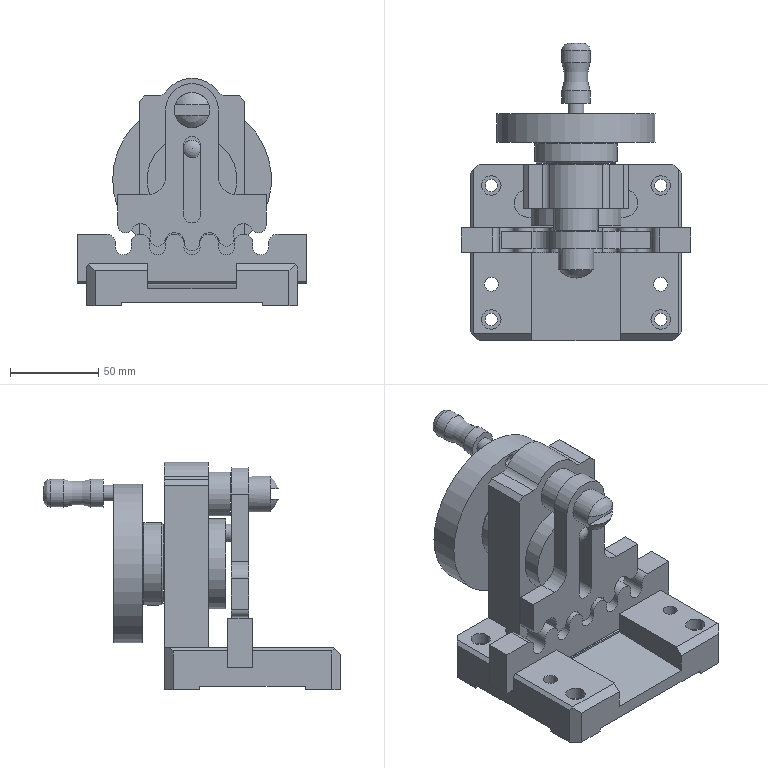Assembly | NX | mm | 15 component files | 15 solids | 303 faces | box 130 x 168.5 x 129 mm | volume 564995 mm3 | plane 157 | cylinder 93 | cone 40 | torus 9 | sphere 3 | spline 1 | commonest cylinder face diameters 16 x10 11 x9 10 x8 8 x8 6 x8 7 x7 20 x6 10.6 x6
Bill of materials:
unnamed part 1 | 1 |  | Thick plain cylindrical ring/bushing: solid cylinder with a single concentric through bore.
unnamed part 2 | 1 |  | Flanged stepped shaft: thin circular flange with one off-center small hole, then a cylindrical section with a circumferential round-bottom groove, stepping down to a smaller-diameter end with a chamfered tip and a short flat or step cut near the end.
GB-T70.1-2000,M6x16 | 1 |  | Hexagon Socket Head Cap Screw, GB-T 70.1-2000,M6x16
unnamed part 3 | 1 |  | Rectangular machined plate with chamfered corners, a straight channel across the top, a stepped rectangular pocket/notch area, a bottom relief making raised end pads, and a pattern of about ten through holes, some with counterbores.
unnamed part 4 | 1 |  | Flat circular disc with a central bore that has an edge chamfer or counterbore, three smaller holes evenly spaced around it in a triangle, and one small hole near the outer rim.
unnamed part 5 | 1 |  | Stepped cylindrical pin: larger-diameter body with a domed (spherical) end, stepping down to a smaller-diameter shank with a chamfered end.
GB73-85,M6x12 | 1 |  | Slotted Set Screw, Flat Point, GB 73-85,M6x12
unnamed part 6 | 1 |  | Annular flange/ring with a large central bore, three through holes evenly spaced around it, chamfered outer edges, and a possible small radial or cross hole meeting the bore.
unnamed part 7 | 1 |  | Straight rectangular bar with a row of five evenly spaced round-bottomed slots cut across one long face, giving a wavy profile with rounded crests.
unnamed part 8 | 1 |  | Rectangular block with an arched raised boss along the top edge, a large chamfered through bore in the main face, and a small hole in the boss region.
unnamed part 9 | 1 |  | Flat T-shaped plate: an upright arm with a rounded end and a circular hole, a long straight slot along the arm, filleted joins into a wide base, and a scalloped lower edge with rounded lobes and notches.
unnamed part 10 | 1 |  | Revolved part shaped like a handle: a rounded-end knob, a concave waisted middle section, a flat shoulder, and a stepped shank made of several smaller cylinders, including a reduced neck.
GB-T70.1-2000,M6x20 | 2 |  | Hexagon Socket Head Cap Screw, GB-T 70.1-2000,M6x20
unnamed part 11 | 1 |  | Stepped pin with a slotted domed head: domed cylindrical head with a straight slot across it, an intermediate cylindrical step, and a long slender cylindrical shank.
Mates:
1. fix | 1_Base_Plate 1 component
2. touch align | 8_Pillar 1 face | 1_Base_Plate 1 face
3. touch align | 8_Pillar 1 face | 1_Base_Plate 1 face
4. touch align | 8_Pillar 1 face | 1_Base_Plate 1 face
5. touch align | 2_Rack 1 face | 1_Base_Plate 1 face
6. center | 2_Rack 1 face | 2_Rack 1 face | 1_Base_Plate 1 face | 1_Base_Plate 1 face
7. center | 6_Balance_Wheel 1 face | 6_Balance_Wheel 1 face | 2_Rack 1 face | 2_Rack 1 face
8. touch align | 6_Balance_Wheel 1 face | 8_Pillar 1 face
9. concentric | 7_Washer 1 edge | 8_Pillar 1 arc
10. concentric | 5_Stud 1 edge | 6_Balance_Wheel 1 edge
11. parallel | 6_Balance_Wheel 1 face | 8_Pillar 1 face
12. concentric | 3_Conn_Shaft 1 edge | 8_Pillar 1 edge
13. concentric | 4_Pin 1 edge | 3_Conn_Shaft 1 edge
14. touch align | 4_Pin 1 face | 6_Balance_Wheel 1 face
15. concentric | 9_Spacer 1 edge | 3_Conn_Shaft 1 edge
16. concentric | 10_Handwheel 1 edge | 9_Spacer 1 edge
17. concentric | 11_Handle 1 edge | 10_Handwheel 1 arc
18. concentric | GB-T70_1-2000_M6x16 1 edge | 10_Handwheel 1 edge
19. concentric | GB-T70_1-2000_M6x20 2 edge | 1_Base_Plate 1 edge
20. concentric | GB-T70_1-2000_M6x20 1 edge | 1_Base_Plate 1 edge
21. touch align | GB73-85_M6x12 1 face | 9_Spacer 1 face
22. touch align | GB73-85_M6x12 1 face | 9_Spacer 1 face